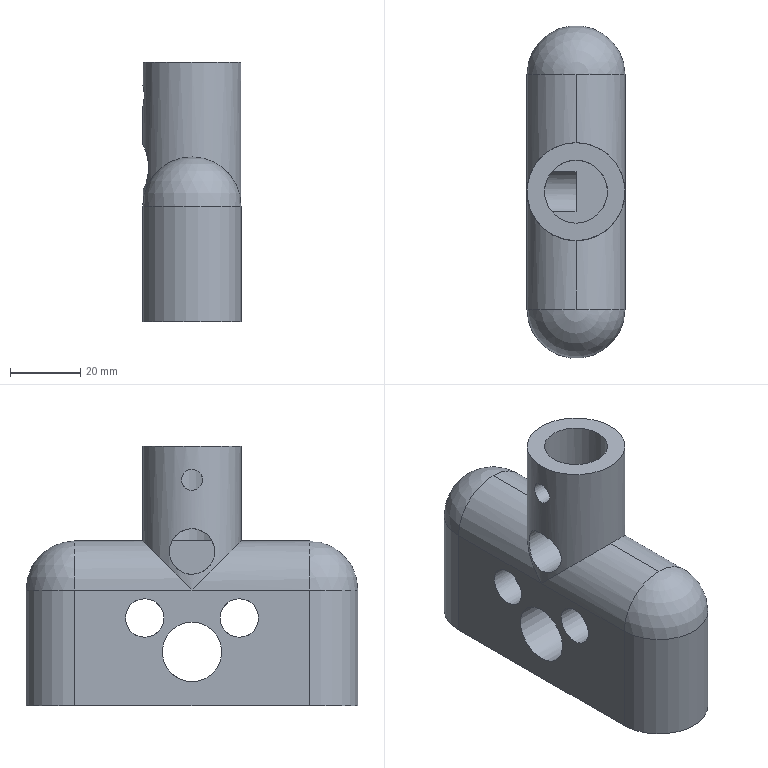Component | NX | UPPER_CYLINDER_BODY | 1 solid | 34 faces | volume 85093 mm3 | cylinder 20 | plane 12 | sphere 2 | commonest cylinder face diameters 28 x7 13 x7 11 x2 17 x1 18 x1 6 x1 8 x1